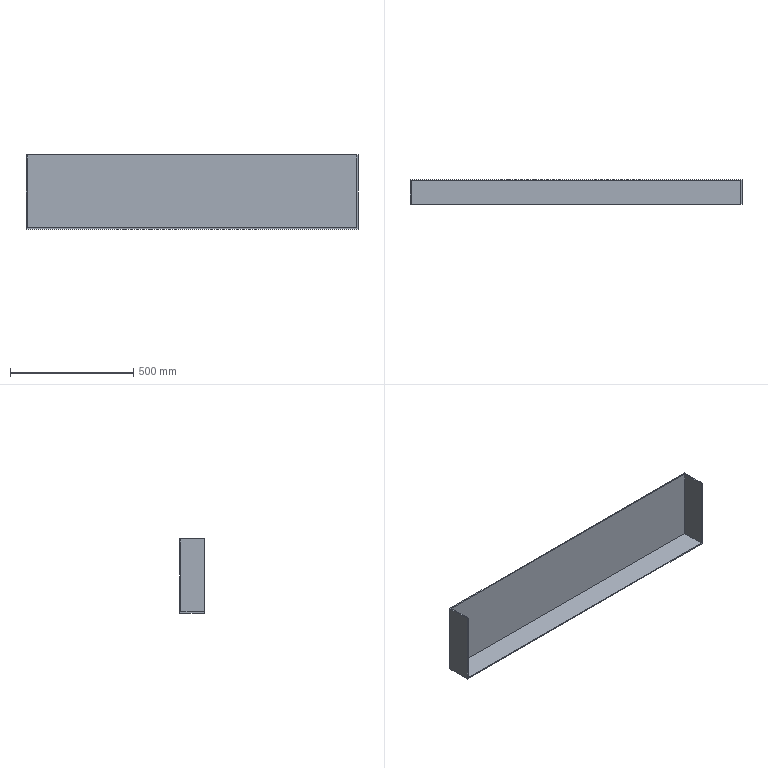Component | SolidWorks | Cover-1 | 1 solid | 10 faces | box 1345 x 100 x 300 mm | volume 2936625 mm3 | plane 10
build123d program:
from build123d import *

# Parameters (mm, degrees)
SKETCH1_W           = 1345
SKETCH1_H           = 300
BOSS_EXTRUDE1_DEPTH = 50
SHELL1_T            = -5


with BuildPart() as part:
    # Sketch1 → Boss-Extrude1 (new, symmetric)
    with BuildSketch(Plane(origin=(0, 0, 0), x_dir=(1, 0, 0), z_dir=(0, 1, 0))):
        Rectangle(SKETCH1_W, SKETCH1_H)
    extrude(amount=BOSS_EXTRUDE1_DEPTH, both=True)

    # Shell1
    shell1_openings = [part.faces().sort_by_distance(p)[0] for p in [
        (0, -50, 0),
        (0, 0, 150),
    ]]
    offset(amount=SHELL1_T, openings=shell1_openings, kind=Kind.INTERSECTION)


solid = part.part

# Placed as in the assembly
solid = solid.moved(Location((0, 672.5, -22.5), (0, 0, 0)))
STEP:
#1=COLOUR_RGB('',0.7922,0.8196,0.9333);
#2=FILL_AREA_STYLE_COLOUR('',#1);
#3=FILL_AREA_STYLE('',(#2));
#4=SURFACE_STYLE_FILL_AREA(#3);
#5=SURFACE_SIDE_STYLE('',(#4));
#6=SURFACE_STYLE_USAGE(.BOTH.,#5);
#7=PRESENTATION_STYLE_ASSIGNMENT((#6));
#8=CARTESIAN_POINT('',(26.28,24.508,5.02));
#9=VERTEX_POINT('',#8);
#10=CARTESIAN_POINT('',(26.476,24.508,5.02));
#11=VERTEX_POINT('',#10);
#12=CARTESIAN_POINT('',(-26.476,24.508,5.02));
#13=DIRECTION('',(1.,0.,0.));
#14=VECTOR('',#13,39.37);
#15=LINE('',#12,#14);
#16=EDGE_CURVE('',#9,#11,#15,.T.);
#17=ORIENTED_EDGE('',*,*,#16,.F.);
#18=CARTESIAN_POINT('',(26.28,24.508,-6.594));
#19=VERTEX_POINT('',#18);
#20=CARTESIAN_POINT('',(26.28,24.508,-0.8858));
#21=DIRECTION('',(0.,0.,-1.));
#22=VECTOR('',#21,39.37);
#23=LINE('',#20,#22);
#24=EDGE_CURVE('',#9,#19,#23,.T.);
#25=ORIENTED_EDGE('',*,*,#24,.T.);
#26=CARTESIAN_POINT('',(-26.28,24.508,-6.594));
#27=VERTEX_POINT('',#26);
#28=CARTESIAN_POINT('',(-0.,24.508,-6.594));
#29=DIRECTION('',(-1.,0.,0.));
#30=VECTOR('',#29,39.37);
#31=LINE('',#28,#30);
#32=EDGE_CURVE('',#19,#27,#31,.T.);
#33=ORIENTED_EDGE('',*,*,#32,.T.);
#34=CARTESIAN_POINT('',(-26.28,24.508,5.02));
#35=VERTEX_POINT('',#34);
#36=CARTESIAN_POINT('',(-26.28,24.508,-0.8858));
#37=DIRECTION('',(0.,0.,1.));
#38=VECTOR('',#37,39.37);
#39=LINE('',#36,#38);
#40=EDGE_CURVE('',#27,#35,#39,.T.);
#41=ORIENTED_EDGE('',*,*,#40,.T.);
#42=CARTESIAN_POINT('',(-26.476,24.508,5.02));
#43=VERTEX_POINT('',#42);
#44=CARTESIAN_POINT('',(-26.476,24.508,5.02));
#45=DIRECTION('',(1.,0.,0.));
#46=VECTOR('',#45,39.37);
#47=LINE('',#44,#46);
#48=EDGE_CURVE('',#43,#35,#47,.T.);
#49=ORIENTED_EDGE('',*,*,#48,.F.);
#50=CARTESIAN_POINT('',(-26.476,24.508,-6.791));
#51=VERTEX_POINT('',#50);
#52=CARTESIAN_POINT('',(-26.476,24.508,5.02));
#53=DIRECTION('',(0.,0.,1.));
#54=VECTOR('',#53,39.37);
#55=LINE('',#52,#54);
#56=EDGE_CURVE('',#51,#43,#55,.T.);
#57=ORIENTED_EDGE('',*,*,#56,.F.);
#58=CARTESIAN_POINT('',(26.476,24.508,-6.791));
#59=VERTEX_POINT('',#58);
#60=CARTESIAN_POINT('',(-26.476,24.508,-6.791));
#61=DIRECTION('',(-1.,0.,0.));
#62=VECTOR('',#61,39.37);
#63=LINE('',#60,#62);
#64=EDGE_CURVE('',#59,#51,#63,.T.);
#65=ORIENTED_EDGE('',*,*,#64,.F.);
#66=CARTESIAN_POINT('',(26.476,24.508,5.02));
#67=DIRECTION('',(0.,0.,-1.));
#68=VECTOR('',#67,39.37);
#69=LINE('',#66,#68);
#70=EDGE_CURVE('',#11,#59,#69,.T.);
#71=ORIENTED_EDGE('',*,*,#70,.F.);
#72=EDGE_LOOP('',(#17,#25,#33,#41,#49,#57,#65,#71));
#73=FACE_OUTER_BOUND('',#72,.T.);
#74=CARTESIAN_POINT('',(-0.,24.508,-0.8858));
#75=DIRECTION('',(0.,-1.,0.));
#76=DIRECTION('',(0.,0.,-1.));
#77=AXIS2_PLACEMENT_3D('',#74,#75,#76);
#78=PLANE('',#77);
#79=ADVANCED_FACE('',(#73),#78,.T.);
#80=ORIENTED_EDGE('',*,*,#70,.T.);
#81=CARTESIAN_POINT('',(26.476,28.445,-6.791));
#82=VERTEX_POINT('',#81);
#83=CARTESIAN_POINT('',(26.476,28.445,-6.791));
#84=DIRECTION('',(0.,-1.,0.));
#85=VECTOR('',#84,39.37);
#86=LINE('',#83,#85);
#87=EDGE_CURVE('',#82,#59,#86,.T.);
#88=ORIENTED_EDGE('',*,*,#87,.F.);
#89=CARTESIAN_POINT('',(26.476,28.445,5.02));
#90=VERTEX_POINT('',#89);
#91=CARTESIAN_POINT('',(26.476,28.445,5.02));
#92=DIRECTION('',(0.,0.,-1.));
#93=VECTOR('',#92,39.37);
#94=LINE('',#91,#93);
#95=EDGE_CURVE('',#90,#82,#94,.T.);
#96=ORIENTED_EDGE('',*,*,#95,.F.);
#97=CARTESIAN_POINT('',(26.476,28.445,5.02));
#98=DIRECTION('',(0.,-1.,0.));
#99=VECTOR('',#98,39.37);
#100=LINE('',#97,#99);
#101=EDGE_CURVE('',#90,#11,#100,.T.);
#102=ORIENTED_EDGE('',*,*,#101,.T.);
#103=EDGE_LOOP('',(#80,#88,#96,#102));
#104=FACE_OUTER_BOUND('',#103,.T.);
#105=CARTESIAN_POINT('',(26.476,28.445,5.02));
#106=DIRECTION('',(-1.,0.,0.));
#107=DIRECTION('',(0.,0.,1.));
#108=AXIS2_PLACEMENT_3D('',#105,#106,#107);
#109=PLANE('',#108);
#110=ADVANCED_FACE('',(#104),#109,.F.);
#111=ORIENTED_EDGE('',*,*,#64,.T.);
#112=CARTESIAN_POINT('',(-26.476,28.445,-6.791));
#113=VERTEX_POINT('',#112);
#114=CARTESIAN_POINT('',(-26.476,28.445,-6.791));
#115=DIRECTION('',(0.,-1.,0.));
#116=VECTOR('',#115,39.37);
#117=LINE('',#114,#116);
#118=EDGE_CURVE('',#113,#51,#117,.T.);
#119=ORIENTED_EDGE('',*,*,#118,.F.);
#120=CARTESIAN_POINT('',(-26.476,28.445,-6.791));
#121=DIRECTION('',(-1.,0.,0.));
#122=VECTOR('',#121,39.37);
#123=LINE('',#120,#122);
#124=EDGE_CURVE('',#82,#113,#123,.T.);
#125=ORIENTED_EDGE('',*,*,#124,.F.);
#126=ORIENTED_EDGE('',*,*,#87,.T.);
#127=EDGE_LOOP('',(#111,#119,#125,#126));
#128=FACE_OUTER_BOUND('',#127,.T.);
#129=CARTESIAN_POINT('',(-26.476,28.445,-6.791));
#130=DIRECTION('',(0.,0.,1.));
#131=DIRECTION('',(1.,0.,0.));
#132=AXIS2_PLACEMENT_3D('',#129,#130,#131);
#133=PLANE('',#132);
#134=ADVANCED_FACE('',(#128),#133,.F.);
#135=ORIENTED_EDGE('',*,*,#56,.T.);
#136=CARTESIAN_POINT('',(-26.476,28.445,5.02));
#137=VERTEX_POINT('',#136);
#138=CARTESIAN_POINT('',(-26.476,28.445,5.02));
#139=DIRECTION('',(0.,-1.,0.));
#140=VECTOR('',#139,39.37);
#141=LINE('',#138,#140);
#142=EDGE_CURVE('',#137,#43,#141,.T.);
#143=ORIENTED_EDGE('',*,*,#142,.F.);
#144=CARTESIAN_POINT('',(-26.476,28.445,5.02));
#145=DIRECTION('',(0.,0.,1.));
#146=VECTOR('',#145,39.37);
#147=LINE('',#144,#146);
#148=EDGE_CURVE('',#113,#137,#147,.T.);
#149=ORIENTED_EDGE('',*,*,#148,.F.);
#150=ORIENTED_EDGE('',*,*,#118,.T.);
#151=EDGE_LOOP('',(#135,#143,#149,#150));
#152=FACE_OUTER_BOUND('',#151,.T.);
#153=CARTESIAN_POINT('',(-26.476,28.445,5.02));
#154=DIRECTION('',(1.,0.,0.));
#155=DIRECTION('',(0.,0.,-1.));
#156=AXIS2_PLACEMENT_3D('',#153,#154,#155);
#157=PLANE('',#156);
#158=ADVANCED_FACE('',(#152),#157,.F.);
#159=CARTESIAN_POINT('',(-26.28,28.248,5.02));
#160=VERTEX_POINT('',#159);
#161=CARTESIAN_POINT('',(26.28,28.248,5.02));
#162=VERTEX_POINT('',#161);
#163=CARTESIAN_POINT('',(-0.,28.248,5.02));
#164=DIRECTION('',(1.,0.,0.));
#165=VECTOR('',#164,39.37);
#166=LINE('',#163,#165);
#167=EDGE_CURVE('',#160,#162,#166,.T.);
#168=ORIENTED_EDGE('',*,*,#167,.T.);
#169=CARTESIAN_POINT('',(26.28,28.445,5.02));
#170=DIRECTION('',(0.,-1.,0.));
#171=VECTOR('',#170,39.37);
#172=LINE('',#169,#171);
#173=EDGE_CURVE('',#162,#9,#172,.T.);
#174=ORIENTED_EDGE('',*,*,#173,.T.);
#175=ORIENTED_EDGE('',*,*,#16,.T.);
#176=ORIENTED_EDGE('',*,*,#101,.F.);
#177=CARTESIAN_POINT('',(-26.476,28.445,5.02));
#178=DIRECTION('',(1.,0.,0.));
#179=VECTOR('',#178,39.37);
#180=LINE('',#177,#179);
#181=EDGE_CURVE('',#137,#90,#180,.T.);
#182=ORIENTED_EDGE('',*,*,#181,.F.);
#183=ORIENTED_EDGE('',*,*,#142,.T.);
#184=ORIENTED_EDGE('',*,*,#48,.T.);
#185=CARTESIAN_POINT('',(-26.28,28.445,5.02));
#186=DIRECTION('',(0.,-1.,0.));
#187=VECTOR('',#186,39.37);
#188=LINE('',#185,#187);
#189=EDGE_CURVE('',#160,#35,#188,.T.);
#190=ORIENTED_EDGE('',*,*,#189,.F.);
#191=EDGE_LOOP('',(#168,#174,#175,#176,#182,#183,#184,#190));
#192=FACE_OUTER_BOUND('',#191,.T.);
#193=CARTESIAN_POINT('',(-26.476,28.445,5.02));
#194=DIRECTION('',(0.,0.,-1.));
#195=DIRECTION('',(-1.,0.,0.));
#196=AXIS2_PLACEMENT_3D('',#193,#194,#195);
#197=PLANE('',#196);
#198=ADVANCED_FACE('',(#192),#197,.F.);
#199=ORIENTED_EDGE('',*,*,#95,.T.);
#200=ORIENTED_EDGE('',*,*,#124,.T.);
#201=ORIENTED_EDGE('',*,*,#148,.T.);
#202=ORIENTED_EDGE('',*,*,#181,.T.);
#203=EDGE_LOOP('',(#199,#200,#201,#202));
#204=FACE_OUTER_BOUND('',#203,.T.);
#205=CARTESIAN_POINT('',(-0.,28.445,-0.8858));
#206=DIRECTION('',(0.,-1.,0.));
#207=DIRECTION('',(0.,0.,-1.));
#208=AXIS2_PLACEMENT_3D('',#205,#206,#207);
#209=PLANE('',#208);
#210=ADVANCED_FACE('',(#204),#209,.F.);
#211=ORIENTED_EDGE('',*,*,#24,.F.);
#212=ORIENTED_EDGE('',*,*,#173,.F.);
#213=CARTESIAN_POINT('',(26.28,28.248,-6.594));
#214=VERTEX_POINT('',#213);
#215=CARTESIAN_POINT('',(26.28,28.248,-0.8858));
#216=DIRECTION('',(0.,0.,-1.));
#217=VECTOR('',#216,39.37);
#218=LINE('',#215,#217);
#219=EDGE_CURVE('',#162,#214,#218,.T.);
#220=ORIENTED_EDGE('',*,*,#219,.T.);
#221=CARTESIAN_POINT('',(26.28,28.445,-6.594));
#222=DIRECTION('',(0.,-1.,0.));
#223=VECTOR('',#222,39.37);
#224=LINE('',#221,#223);
#225=EDGE_CURVE('',#214,#19,#224,.T.);
#226=ORIENTED_EDGE('',*,*,#225,.T.);
#227=EDGE_LOOP('',(#211,#212,#220,#226));
#228=FACE_OUTER_BOUND('',#227,.T.);
#229=CARTESIAN_POINT('',(26.28,28.445,5.02));
#230=DIRECTION('',(-1.,0.,0.));
#231=DIRECTION('',(0.,0.,1.));
#232=AXIS2_PLACEMENT_3D('',#229,#230,#231);
#233=PLANE('',#232);
#234=ADVANCED_FACE('',(#228),#233,.T.);
#235=ORIENTED_EDGE('',*,*,#32,.F.);
#236=ORIENTED_EDGE('',*,*,#225,.F.);
#237=CARTESIAN_POINT('',(-26.28,28.248,-6.594));
#238=VERTEX_POINT('',#237);
#239=CARTESIAN_POINT('',(-0.,28.248,-6.594));
#240=DIRECTION('',(-1.,0.,0.));
#241=VECTOR('',#240,39.37);
#242=LINE('',#239,#241);
#243=EDGE_CURVE('',#214,#238,#242,.T.);
#244=ORIENTED_EDGE('',*,*,#243,.T.);
#245=CARTESIAN_POINT('',(-26.28,28.445,-6.594));
#246=DIRECTION('',(0.,-1.,0.));
#247=VECTOR('',#246,39.37);
#248=LINE('',#245,#247);
#249=EDGE_CURVE('',#238,#27,#248,.T.);
#250=ORIENTED_EDGE('',*,*,#249,.T.);
#251=EDGE_LOOP('',(#235,#236,#244,#250));
#252=FACE_OUTER_BOUND('',#251,.T.);
#253=CARTESIAN_POINT('',(-26.476,28.445,-6.594));
#254=DIRECTION('',(0.,0.,1.));
#255=DIRECTION('',(1.,0.,0.));
#256=AXIS2_PLACEMENT_3D('',#253,#254,#255);
#257=PLANE('',#256);
#258=ADVANCED_FACE('',(#252),#257,.T.);
#259=ORIENTED_EDGE('',*,*,#40,.F.);
#260=ORIENTED_EDGE('',*,*,#249,.F.);
#261=CARTESIAN_POINT('',(-26.28,28.248,-0.8858));
#262=DIRECTION('',(0.,0.,1.));
#263=VECTOR('',#262,39.37);
#264=LINE('',#261,#263);
#265=EDGE_CURVE('',#238,#160,#264,.T.);
#266=ORIENTED_EDGE('',*,*,#265,.T.);
#267=ORIENTED_EDGE('',*,*,#189,.T.);
#268=EDGE_LOOP('',(#259,#260,#266,#267));
#269=FACE_OUTER_BOUND('',#268,.T.);
#270=CARTESIAN_POINT('',(-26.28,28.445,5.02));
#271=DIRECTION('',(1.,0.,0.));
#272=DIRECTION('',(0.,0.,-1.));
#273=AXIS2_PLACEMENT_3D('',#270,#271,#272);
#274=PLANE('',#273);
#275=ADVANCED_FACE('',(#269),#274,.T.);
#276=ORIENTED_EDGE('',*,*,#219,.F.);
#277=ORIENTED_EDGE('',*,*,#167,.F.);
#278=ORIENTED_EDGE('',*,*,#265,.F.);
#279=ORIENTED_EDGE('',*,*,#243,.F.);
#280=EDGE_LOOP('',(#276,#277,#278,#279));
#281=FACE_OUTER_BOUND('',#280,.T.);
#282=CARTESIAN_POINT('',(-0.,28.248,-0.8858));
#283=DIRECTION('',(0.,-1.,0.));
#284=DIRECTION('',(0.,0.,-1.));
#285=AXIS2_PLACEMENT_3D('',#282,#283,#284);
#286=PLANE('',#285);
#287=ADVANCED_FACE('',(#281),#286,.T.);
#288=CLOSED_SHELL('',(#79,#110,#134,#158,#198,#210,#234,#258,#275,#287));
#289=MANIFOLD_SOLID_BREP('',#288);
#290=STYLED_ITEM('',(#7),#289);
#291=(LENGTH_UNIT()NAMED_UNIT(*)SI_UNIT($,.METRE.));
#292=LENGTH_MEASURE_WITH_UNIT(LENGTH_MEASURE(0.0254),#291);
#293=DIMENSIONAL_EXPONENTS(1.,0.,0.,0.,0.,0.,0.);
#294=(CONVERSION_BASED_UNIT('',#292)LENGTH_UNIT()NAMED_UNIT(#293));
#295=UNCERTAINTY_MEASURE_WITH_UNIT(LENGTH_MEASURE(0.00001),#294,'','');
#296=(NAMED_UNIT(*)PLANE_ANGLE_UNIT()SI_UNIT($,.RADIAN.));
#297=(NAMED_UNIT(*)SI_UNIT($,.STERADIAN.)SOLID_ANGLE_UNIT());
#298=(GEOMETRIC_REPRESENTATION_CONTEXT(3)GLOBAL_UNCERTAINTY_ASSIGNED_CONTEXT((#295))GLOBAL_UNIT_ASSIGNED_CONTEXT((#294,#296,#297))REPRESENTATION_CONTEXT('',''));
#299=MECHANICAL_DESIGN_GEOMETRIC_PRESENTATION_REPRESENTATION('',(#290),#298);
#300=PRESENTATION_LAYER_ASSIGNMENT('','',(#290));
#301=CARTESIAN_POINT('',(0.,0.,0.));
#302=DIRECTION('',(0.,0.,1.));
#303=DIRECTION('',(1.,0.,0.));
#304=AXIS2_PLACEMENT_3D('',#301,#302,#303);
#305=(LENGTH_UNIT()NAMED_UNIT(*)SI_UNIT($,.METRE.));
#306=LENGTH_MEASURE_WITH_UNIT(LENGTH_MEASURE(0.0254),#305);
#307=DIMENSIONAL_EXPONENTS(1.,0.,0.,0.,0.,0.,0.);
#308=(CONVERSION_BASED_UNIT('',#306)LENGTH_UNIT()NAMED_UNIT(#307));
#309=UNCERTAINTY_MEASURE_WITH_UNIT(LENGTH_MEASURE(0.00001),#308,'','');
#310=(NAMED_UNIT(*)PLANE_ANGLE_UNIT()SI_UNIT($,.RADIAN.));
#311=(NAMED_UNIT(*)SI_UNIT($,.STERADIAN.)SOLID_ANGLE_UNIT());
#312=(GEOMETRIC_REPRESENTATION_CONTEXT(3)GLOBAL_UNCERTAINTY_ASSIGNED_CONTEXT((#309))GLOBAL_UNIT_ASSIGNED_CONTEXT((#308,#310,#311))REPRESENTATION_CONTEXT('',''));
#313=ADVANCED_BREP_SHAPE_REPRESENTATION('',(#289,#304),#312);